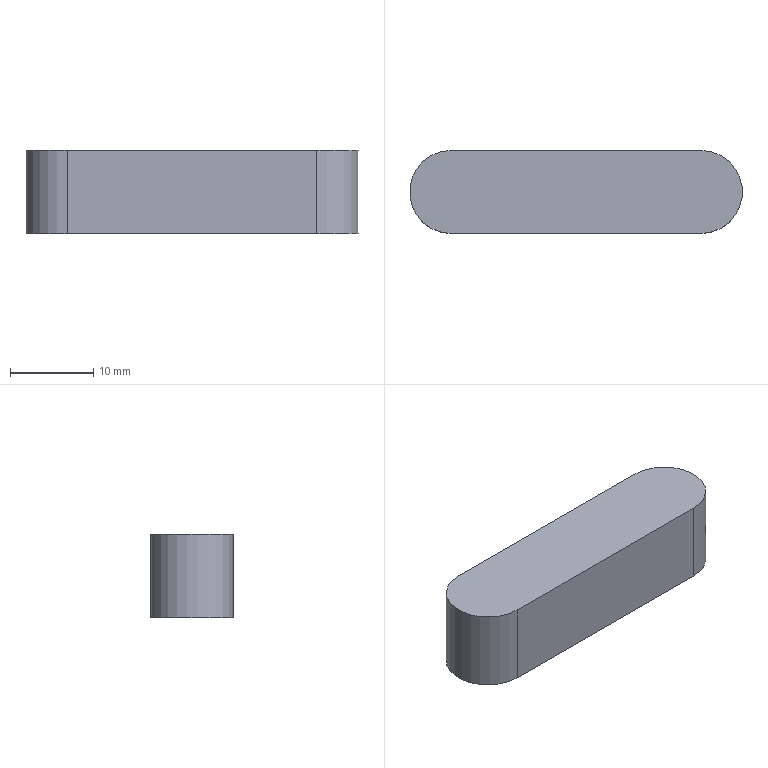Component | NX | PINGJIAN10 | 1 solid | 6 faces | box 40 x 10 x 10 mm | volume 3785 mm3 | plane 4 | cylinder 2 | commonest cylinder face diameters 10 x2
STEP:
#1=CARTESIAN_POINT('',(0.,0.,0.));
#2=DIRECTION('',(0.,0.,1.));
#3=DIRECTION('',(1.,0.,0.));
#4=AXIS2_PLACEMENT_3D('',#1,#2,#3);
#5=CARTESIAN_POINT('',(15.25,205.,-68.));
#6=VERTEX_POINT('',#5);
#7=CARTESIAN_POINT('',(15.25,195.,-68.));
#8=VERTEX_POINT('',#7);
#9=CARTESIAN_POINT('',(15.25,200.,-68.));
#10=DIRECTION('',(0.,0.,1.));
#11=DIRECTION('',(1.,0.,0.));
#12=AXIS2_PLACEMENT_3D('',#9,#10,#11);
#13=CIRCLE('',#12,5.);
#14=CARTESIAN_POINT('',(15.25,200.,-58.));
#15=DIRECTION('',(0.,0.,-1.));
#16=DIRECTION('',(-1.,0.,0.));
#17=AXIS2_PLACEMENT_3D('',#14,#15,#16);
#18=CYLINDRICAL_SURFACE('',#17,5.);
#19=CARTESIAN_POINT('',(3.142,10.));
#20=DIRECTION('',(-1.,0.));
#21=VECTOR('',#20,1.);
#22=LINE('',#19,#21);
#23=(GEOMETRIC_REPRESENTATION_CONTEXT(2)PARAMETRIC_REPRESENTATION_CONTEXT()REPRESENTATION_CONTEXT('',''));
#24=DEFINITIONAL_REPRESENTATION('',(#22),#23);
#25=PCURVE('',#18,#24);
#26=CARTESIAN_POINT('',(15.25,200.,-68.));
#27=DIRECTION('',(0.,0.,1.));
#28=DIRECTION('',(1.,0.,0.));
#29=AXIS2_PLACEMENT_3D('',#26,#27,#28);
#30=PLANE('',#29);
#31=CARTESIAN_POINT('',(0.,0.));
#32=DIRECTION('',(1.,0.));
#33=AXIS2_PLACEMENT_2D('',#31,#32);
#34=CIRCLE('',#33,5.);
#35=(GEOMETRIC_REPRESENTATION_CONTEXT(2)PARAMETRIC_REPRESENTATION_CONTEXT()REPRESENTATION_CONTEXT('',''));
#36=DEFINITIONAL_REPRESENTATION('',(#34),#35);
#37=PCURVE('',#30,#36);
#38=SURFACE_CURVE('',#13,(#25,#37),.PCURVE_S1.);
#39=EDGE_CURVE('',#6,#8,#38,.T.);
#40=ORIENTED_EDGE('',*,*,#39,.T.);
#41=CARTESIAN_POINT('',(15.25,195.,-58.));
#42=VERTEX_POINT('',#41);
#43=CARTESIAN_POINT('',(15.25,195.,-58.));
#44=DIRECTION('',(0.,0.,-1.));
#45=VECTOR('',#44,1.);
#46=LINE('',#43,#45);
#47=CARTESIAN_POINT('',(-1.571,0.));
#48=DIRECTION('',(0.,1.));
#49=VECTOR('',#48,1.);
#50=LINE('',#47,#49);
#51=(GEOMETRIC_REPRESENTATION_CONTEXT(2)PARAMETRIC_REPRESENTATION_CONTEXT()REPRESENTATION_CONTEXT('',''));
#52=DEFINITIONAL_REPRESENTATION('',(#50),#51);
#53=PCURVE('',#18,#52);
#54=CARTESIAN_POINT('',(15.25,195.,-58.));
#55=DIRECTION('',(0.,1.,0.));
#56=DIRECTION('',(0.,0.,1.));
#57=AXIS2_PLACEMENT_3D('',#54,#55,#56);
#58=PLANE('',#57);
#59=CARTESIAN_POINT('',(0.,0.));
#60=DIRECTION('',(-1.,0.));
#61=VECTOR('',#60,1.);
#62=LINE('',#59,#61);
#63=(GEOMETRIC_REPRESENTATION_CONTEXT(2)PARAMETRIC_REPRESENTATION_CONTEXT()REPRESENTATION_CONTEXT('',''));
#64=DEFINITIONAL_REPRESENTATION('',(#62),#63);
#65=PCURVE('',#58,#64);
#66=SURFACE_CURVE('',#46,(#53,#65),.PCURVE_S1.);
#67=EDGE_CURVE('',#42,#8,#66,.T.);
#68=ORIENTED_EDGE('',*,*,#67,.F.);
#69=CARTESIAN_POINT('',(15.25,205.,-58.));
#70=VERTEX_POINT('',#69);
#71=CARTESIAN_POINT('',(15.25,200.,-58.));
#72=DIRECTION('',(0.,0.,1.));
#73=DIRECTION('',(1.,0.,0.));
#74=AXIS2_PLACEMENT_3D('',#71,#72,#73);
#75=CIRCLE('',#74,5.);
#76=CARTESIAN_POINT('',(3.142,0.));
#77=DIRECTION('',(-1.,0.));
#78=VECTOR('',#77,1.);
#79=LINE('',#76,#78);
#80=(GEOMETRIC_REPRESENTATION_CONTEXT(2)PARAMETRIC_REPRESENTATION_CONTEXT()REPRESENTATION_CONTEXT('',''));
#81=DEFINITIONAL_REPRESENTATION('',(#79),#80);
#82=PCURVE('',#18,#81);
#83=CARTESIAN_POINT('',(15.25,200.,-58.));
#84=DIRECTION('',(0.,0.,1.));
#85=DIRECTION('',(1.,0.,0.));
#86=AXIS2_PLACEMENT_3D('',#83,#84,#85);
#87=PLANE('',#86);
#88=CARTESIAN_POINT('',(0.,0.));
#89=DIRECTION('',(1.,0.));
#90=AXIS2_PLACEMENT_2D('',#88,#89);
#91=CIRCLE('',#90,5.);
#92=(GEOMETRIC_REPRESENTATION_CONTEXT(2)PARAMETRIC_REPRESENTATION_CONTEXT()REPRESENTATION_CONTEXT('',''));
#93=DEFINITIONAL_REPRESENTATION('',(#91),#92);
#94=PCURVE('',#87,#93);
#95=SURFACE_CURVE('',#75,(#82,#94),.PCURVE_S1.);
#96=EDGE_CURVE('',#70,#42,#95,.T.);
#97=ORIENTED_EDGE('',*,*,#96,.F.);
#98=CARTESIAN_POINT('',(15.25,205.,-58.));
#99=DIRECTION('',(0.,0.,-1.));
#100=VECTOR('',#99,1.);
#101=LINE('',#98,#100);
#102=CARTESIAN_POINT('',(1.571,0.));
#103=DIRECTION('',(0.,1.));
#104=VECTOR('',#103,1.);
#105=LINE('',#102,#104);
#106=(GEOMETRIC_REPRESENTATION_CONTEXT(2)PARAMETRIC_REPRESENTATION_CONTEXT()REPRESENTATION_CONTEXT('',''));
#107=DEFINITIONAL_REPRESENTATION('',(#105),#106);
#108=PCURVE('',#18,#107);
#109=CARTESIAN_POINT('',(45.25,205.,-58.));
#110=DIRECTION('',(0.,-1.,0.));
#111=DIRECTION('',(0.,0.,-1.));
#112=AXIS2_PLACEMENT_3D('',#109,#110,#111);
#113=PLANE('',#112);
#114=CARTESIAN_POINT('',(0.,-30.));
#115=DIRECTION('',(1.,0.));
#116=VECTOR('',#115,1.);
#117=LINE('',#114,#116);
#118=(GEOMETRIC_REPRESENTATION_CONTEXT(2)PARAMETRIC_REPRESENTATION_CONTEXT()REPRESENTATION_CONTEXT('',''));
#119=DEFINITIONAL_REPRESENTATION('',(#117),#118);
#120=PCURVE('',#113,#119);
#121=SURFACE_CURVE('',#101,(#108,#120),.PCURVE_S1.);
#122=EDGE_CURVE('',#70,#6,#121,.T.);
#123=ORIENTED_EDGE('',*,*,#122,.T.);
#124=EDGE_LOOP('',(#40,#68,#97,#123));
#125=FACE_BOUND('',#124,.T.);
#126=ADVANCED_FACE('',(#125),#18,.T.);
#127=CARTESIAN_POINT('',(45.25,195.,-68.));
#128=VERTEX_POINT('',#127);
#129=CARTESIAN_POINT('',(15.25,195.,-68.));
#130=DIRECTION('',(1.,0.,0.));
#131=VECTOR('',#130,1.);
#132=LINE('',#129,#131);
#133=CARTESIAN_POINT('',(-10.,0.));
#134=DIRECTION('',(0.,1.));
#135=VECTOR('',#134,1.);
#136=LINE('',#133,#135);
#137=(GEOMETRIC_REPRESENTATION_CONTEXT(2)PARAMETRIC_REPRESENTATION_CONTEXT()REPRESENTATION_CONTEXT('',''));
#138=DEFINITIONAL_REPRESENTATION('',(#136),#137);
#139=PCURVE('',#58,#138);
#140=CARTESIAN_POINT('',(0.,-5.));
#141=DIRECTION('',(1.,0.));
#142=VECTOR('',#141,1.);
#143=LINE('',#140,#142);
#144=(GEOMETRIC_REPRESENTATION_CONTEXT(2)PARAMETRIC_REPRESENTATION_CONTEXT()REPRESENTATION_CONTEXT('',''));
#145=DEFINITIONAL_REPRESENTATION('',(#143),#144);
#146=PCURVE('',#30,#145);
#147=SURFACE_CURVE('',#132,(#139,#146),.PCURVE_S1.);
#148=EDGE_CURVE('',#8,#128,#147,.T.);
#149=ORIENTED_EDGE('',*,*,#148,.T.);
#150=CARTESIAN_POINT('',(45.25,195.,-58.));
#151=VERTEX_POINT('',#150);
#152=CARTESIAN_POINT('',(45.25,195.,-58.));
#153=DIRECTION('',(0.,0.,-1.));
#154=VECTOR('',#153,1.);
#155=LINE('',#152,#154);
#156=CARTESIAN_POINT('',(0.,30.));
#157=DIRECTION('',(-1.,0.));
#158=VECTOR('',#157,1.);
#159=LINE('',#156,#158);
#160=(GEOMETRIC_REPRESENTATION_CONTEXT(2)PARAMETRIC_REPRESENTATION_CONTEXT()REPRESENTATION_CONTEXT('',''));
#161=DEFINITIONAL_REPRESENTATION('',(#159),#160);
#162=PCURVE('',#58,#161);
#163=CARTESIAN_POINT('',(45.25,200.,-58.));
#164=DIRECTION('',(0.,0.,-1.));
#165=DIRECTION('',(-1.,0.,0.));
#166=AXIS2_PLACEMENT_3D('',#163,#164,#165);
#167=CYLINDRICAL_SURFACE('',#166,5.);
#168=CARTESIAN_POINT('',(4.712,0.));
#169=DIRECTION('',(0.,1.));
#170=VECTOR('',#169,1.);
#171=LINE('',#168,#170);
#172=(GEOMETRIC_REPRESENTATION_CONTEXT(2)PARAMETRIC_REPRESENTATION_CONTEXT()REPRESENTATION_CONTEXT('',''));
#173=DEFINITIONAL_REPRESENTATION('',(#171),#172);
#174=PCURVE('',#167,#173);
#175=SURFACE_CURVE('',#155,(#162,#174),.PCURVE_S1.);
#176=EDGE_CURVE('',#151,#128,#175,.T.);
#177=ORIENTED_EDGE('',*,*,#176,.F.);
#178=CARTESIAN_POINT('',(15.25,195.,-58.));
#179=DIRECTION('',(1.,0.,0.));
#180=VECTOR('',#179,1.);
#181=LINE('',#178,#180);
#182=CARTESIAN_POINT('',(0.,0.));
#183=DIRECTION('',(0.,1.));
#184=VECTOR('',#183,1.);
#185=LINE('',#182,#184);
#186=(GEOMETRIC_REPRESENTATION_CONTEXT(2)PARAMETRIC_REPRESENTATION_CONTEXT()REPRESENTATION_CONTEXT('',''));
#187=DEFINITIONAL_REPRESENTATION('',(#185),#186);
#188=PCURVE('',#58,#187);
#189=CARTESIAN_POINT('',(0.,-5.));
#190=DIRECTION('',(1.,0.));
#191=VECTOR('',#190,1.);
#192=LINE('',#189,#191);
#193=(GEOMETRIC_REPRESENTATION_CONTEXT(2)PARAMETRIC_REPRESENTATION_CONTEXT()REPRESENTATION_CONTEXT('',''));
#194=DEFINITIONAL_REPRESENTATION('',(#192),#193);
#195=PCURVE('',#87,#194);
#196=SURFACE_CURVE('',#181,(#188,#195),.PCURVE_S1.);
#197=EDGE_CURVE('',#42,#151,#196,.T.);
#198=ORIENTED_EDGE('',*,*,#197,.F.);
#199=ORIENTED_EDGE('',*,*,#67,.T.);
#200=EDGE_LOOP('',(#149,#177,#198,#199));
#201=FACE_BOUND('',#200,.T.);
#202=ADVANCED_FACE('',(#201),#58,.F.);
#203=CARTESIAN_POINT('',(45.25,205.,-68.));
#204=VERTEX_POINT('',#203);
#205=CARTESIAN_POINT('',(45.25,200.,-68.));
#206=DIRECTION('',(0.,0.,1.));
#207=DIRECTION('',(1.,0.,0.));
#208=AXIS2_PLACEMENT_3D('',#205,#206,#207);
#209=CIRCLE('',#208,5.);
#210=CARTESIAN_POINT('',(9.425,10.));
#211=DIRECTION('',(-1.,0.));
#212=VECTOR('',#211,1.);
#213=LINE('',#210,#212);
#214=(GEOMETRIC_REPRESENTATION_CONTEXT(2)PARAMETRIC_REPRESENTATION_CONTEXT()REPRESENTATION_CONTEXT('',''));
#215=DEFINITIONAL_REPRESENTATION('',(#213),#214);
#216=PCURVE('',#167,#215);
#217=CARTESIAN_POINT('',(30.,0.));
#218=DIRECTION('',(1.,0.));
#219=AXIS2_PLACEMENT_2D('',#217,#218);
#220=CIRCLE('',#219,5.);
#221=(GEOMETRIC_REPRESENTATION_CONTEXT(2)PARAMETRIC_REPRESENTATION_CONTEXT()REPRESENTATION_CONTEXT('',''));
#222=DEFINITIONAL_REPRESENTATION('',(#220),#221);
#223=PCURVE('',#30,#222);
#224=SURFACE_CURVE('',#209,(#216,#223),.PCURVE_S1.);
#225=EDGE_CURVE('',#128,#204,#224,.T.);
#226=ORIENTED_EDGE('',*,*,#225,.T.);
#227=CARTESIAN_POINT('',(45.25,205.,-58.));
#228=VERTEX_POINT('',#227);
#229=CARTESIAN_POINT('',(45.25,205.,-58.));
#230=DIRECTION('',(0.,0.,-1.));
#231=VECTOR('',#230,1.);
#232=LINE('',#229,#231);
#233=CARTESIAN_POINT('',(1.571,0.));
#234=DIRECTION('',(0.,1.));
#235=VECTOR('',#234,1.);
#236=LINE('',#233,#235);
#237=(GEOMETRIC_REPRESENTATION_CONTEXT(2)PARAMETRIC_REPRESENTATION_CONTEXT()REPRESENTATION_CONTEXT('',''));
#238=DEFINITIONAL_REPRESENTATION('',(#236),#237);
#239=PCURVE('',#167,#238);
#240=CARTESIAN_POINT('',(0.,0.));
#241=DIRECTION('',(1.,0.));
#242=VECTOR('',#241,1.);
#243=LINE('',#240,#242);
#244=(GEOMETRIC_REPRESENTATION_CONTEXT(2)PARAMETRIC_REPRESENTATION_CONTEXT()REPRESENTATION_CONTEXT('',''));
#245=DEFINITIONAL_REPRESENTATION('',(#243),#244);
#246=PCURVE('',#113,#245);
#247=SURFACE_CURVE('',#232,(#239,#246),.PCURVE_S1.);
#248=EDGE_CURVE('',#228,#204,#247,.T.);
#249=ORIENTED_EDGE('',*,*,#248,.F.);
#250=CARTESIAN_POINT('',(45.25,200.,-58.));
#251=DIRECTION('',(0.,0.,1.));
#252=DIRECTION('',(1.,0.,0.));
#253=AXIS2_PLACEMENT_3D('',#250,#251,#252);
#254=CIRCLE('',#253,5.);
#255=CARTESIAN_POINT('',(9.425,0.));
#256=DIRECTION('',(-1.,0.));
#257=VECTOR('',#256,1.);
#258=LINE('',#255,#257);
#259=(GEOMETRIC_REPRESENTATION_CONTEXT(2)PARAMETRIC_REPRESENTATION_CONTEXT()REPRESENTATION_CONTEXT('',''));
#260=DEFINITIONAL_REPRESENTATION('',(#258),#259);
#261=PCURVE('',#167,#260);
#262=CARTESIAN_POINT('',(30.,0.));
#263=DIRECTION('',(1.,0.));
#264=AXIS2_PLACEMENT_2D('',#262,#263);
#265=CIRCLE('',#264,5.);
#266=(GEOMETRIC_REPRESENTATION_CONTEXT(2)PARAMETRIC_REPRESENTATION_CONTEXT()REPRESENTATION_CONTEXT('',''));
#267=DEFINITIONAL_REPRESENTATION('',(#265),#266);
#268=PCURVE('',#87,#267);
#269=SURFACE_CURVE('',#254,(#261,#268),.PCURVE_S1.);
#270=EDGE_CURVE('',#151,#228,#269,.T.);
#271=ORIENTED_EDGE('',*,*,#270,.F.);
#272=ORIENTED_EDGE('',*,*,#176,.T.);
#273=EDGE_LOOP('',(#226,#249,#271,#272));
#274=FACE_BOUND('',#273,.T.);
#275=ADVANCED_FACE('',(#274),#167,.T.);
#276=CARTESIAN_POINT('',(45.25,205.,-68.));
#277=DIRECTION('',(-1.,0.,0.));
#278=VECTOR('',#277,1.);
#279=LINE('',#276,#278);
#280=CARTESIAN_POINT('',(10.,0.));
#281=DIRECTION('',(0.,-1.));
#282=VECTOR('',#281,1.);
#283=LINE('',#280,#282);
#284=(GEOMETRIC_REPRESENTATION_CONTEXT(2)PARAMETRIC_REPRESENTATION_CONTEXT()REPRESENTATION_CONTEXT('',''));
#285=DEFINITIONAL_REPRESENTATION('',(#283),#284);
#286=PCURVE('',#113,#285);
#287=CARTESIAN_POINT('',(30.,5.));
#288=DIRECTION('',(-1.,0.));
#289=VECTOR('',#288,1.);
#290=LINE('',#287,#289);
#291=(GEOMETRIC_REPRESENTATION_CONTEXT(2)PARAMETRIC_REPRESENTATION_CONTEXT()REPRESENTATION_CONTEXT('',''));
#292=DEFINITIONAL_REPRESENTATION('',(#290),#291);
#293=PCURVE('',#30,#292);
#294=SURFACE_CURVE('',#279,(#286,#293),.PCURVE_S1.);
#295=EDGE_CURVE('',#204,#6,#294,.T.);
#296=ORIENTED_EDGE('',*,*,#295,.T.);
#297=ORIENTED_EDGE('',*,*,#122,.F.);
#298=CARTESIAN_POINT('',(45.25,205.,-58.));
#299=DIRECTION('',(-1.,0.,0.));
#300=VECTOR('',#299,1.);
#301=LINE('',#298,#300);
#302=CARTESIAN_POINT('',(0.,0.));
#303=DIRECTION('',(0.,-1.));
#304=VECTOR('',#303,1.);
#305=LINE('',#302,#304);
#306=(GEOMETRIC_REPRESENTATION_CONTEXT(2)PARAMETRIC_REPRESENTATION_CONTEXT()REPRESENTATION_CONTEXT('',''));
#307=DEFINITIONAL_REPRESENTATION('',(#305),#306);
#308=PCURVE('',#113,#307);
#309=CARTESIAN_POINT('',(30.,5.));
#310=DIRECTION('',(-1.,0.));
#311=VECTOR('',#310,1.);
#312=LINE('',#309,#311);
#313=(GEOMETRIC_REPRESENTATION_CONTEXT(2)PARAMETRIC_REPRESENTATION_CONTEXT()REPRESENTATION_CONTEXT('',''));
#314=DEFINITIONAL_REPRESENTATION('',(#312),#313);
#315=PCURVE('',#87,#314);
#316=SURFACE_CURVE('',#301,(#308,#315),.PCURVE_S1.);
#317=EDGE_CURVE('',#228,#70,#316,.T.);
#318=ORIENTED_EDGE('',*,*,#317,.F.);
#319=ORIENTED_EDGE('',*,*,#248,.T.);
#320=EDGE_LOOP('',(#296,#297,#318,#319));
#321=FACE_BOUND('',#320,.T.);
#322=ADVANCED_FACE('',(#321),#113,.F.);
#323=ORIENTED_EDGE('',*,*,#96,.T.);
#324=ORIENTED_EDGE('',*,*,#197,.T.);
#325=ORIENTED_EDGE('',*,*,#270,.T.);
#326=ORIENTED_EDGE('',*,*,#317,.T.);
#327=EDGE_LOOP('',(#323,#324,#325,#326));
#328=FACE_BOUND('',#327,.T.);
#329=ADVANCED_FACE('',(#328),#87,.T.);
#330=ORIENTED_EDGE('',*,*,#39,.F.);
#331=ORIENTED_EDGE('',*,*,#295,.F.);
#332=ORIENTED_EDGE('',*,*,#225,.F.);
#333=ORIENTED_EDGE('',*,*,#148,.F.);
#334=EDGE_LOOP('',(#330,#331,#332,#333));
#335=FACE_BOUND('',#334,.T.);
#336=ADVANCED_FACE('',(#335),#30,.F.);
#337=CLOSED_SHELL('',(#126,#202,#275,#322,#329,#336));
#338=MANIFOLD_SOLID_BREP('',#337);
#339=(LENGTH_UNIT()NAMED_UNIT(*)SI_UNIT(.MILLI.,.METRE.));
#340=UNCERTAINTY_MEASURE_WITH_UNIT(LENGTH_MEASURE(0.0000001),#339,'','');
#341=(NAMED_UNIT(*)PLANE_ANGLE_UNIT()SI_UNIT($,.RADIAN.));
#342=(NAMED_UNIT(*)SI_UNIT($,.STERADIAN.)SOLID_ANGLE_UNIT());
#343=(GEOMETRIC_REPRESENTATION_CONTEXT(3)GLOBAL_UNCERTAINTY_ASSIGNED_CONTEXT((#340))GLOBAL_UNIT_ASSIGNED_CONTEXT((#339,#341,#342))REPRESENTATION_CONTEXT('',''));
#344=ADVANCED_BREP_SHAPE_REPRESENTATION('',(#4,#338),#343);